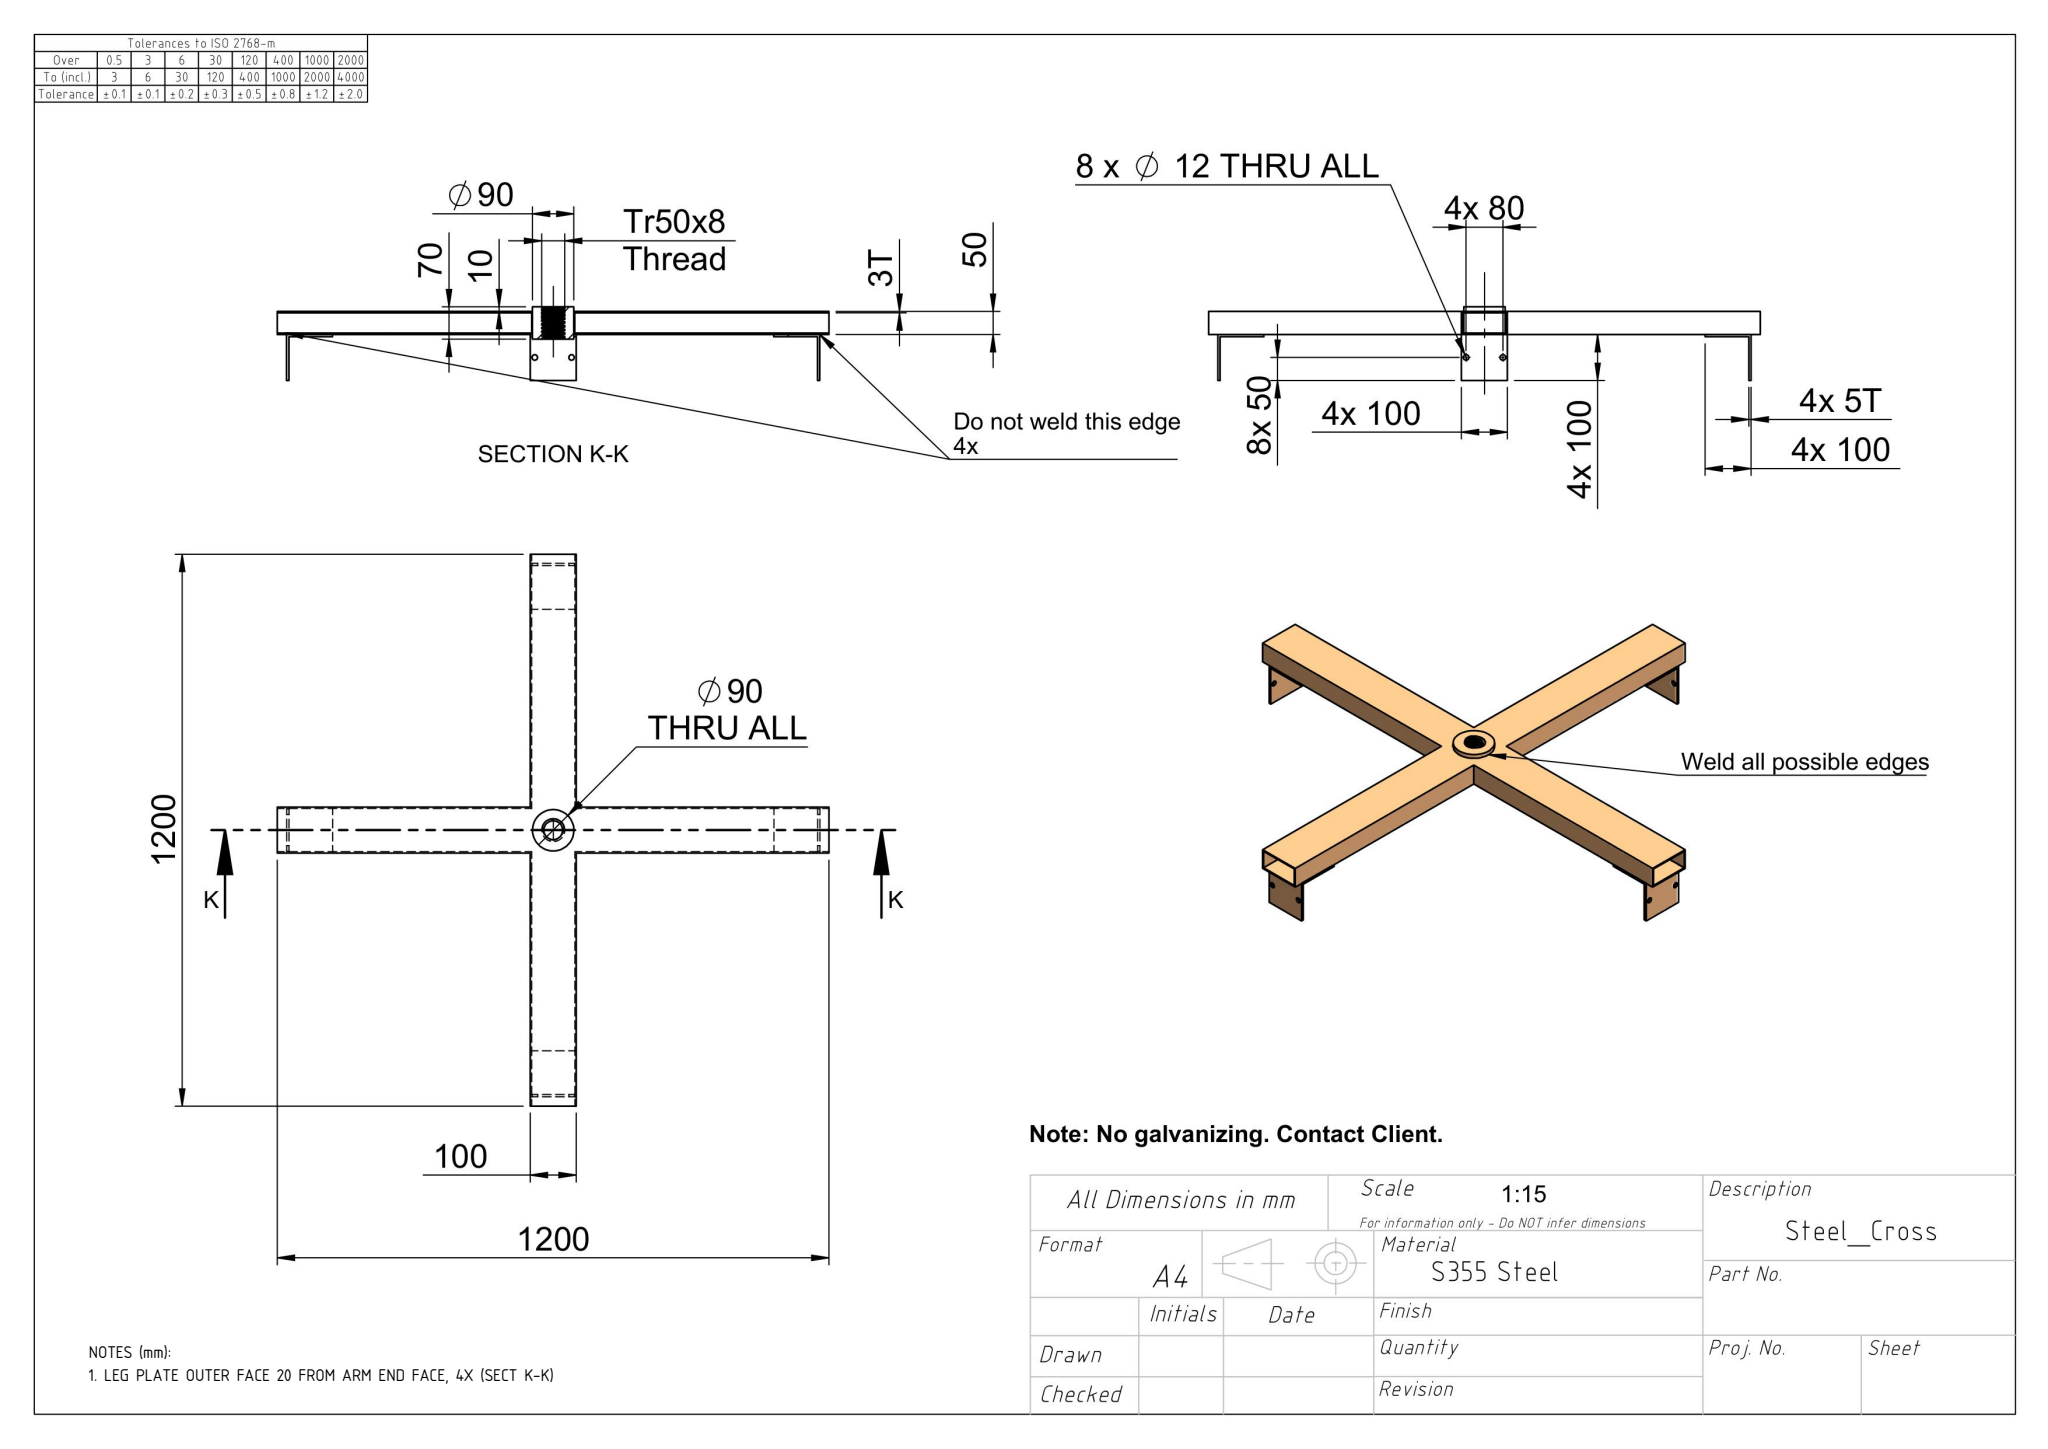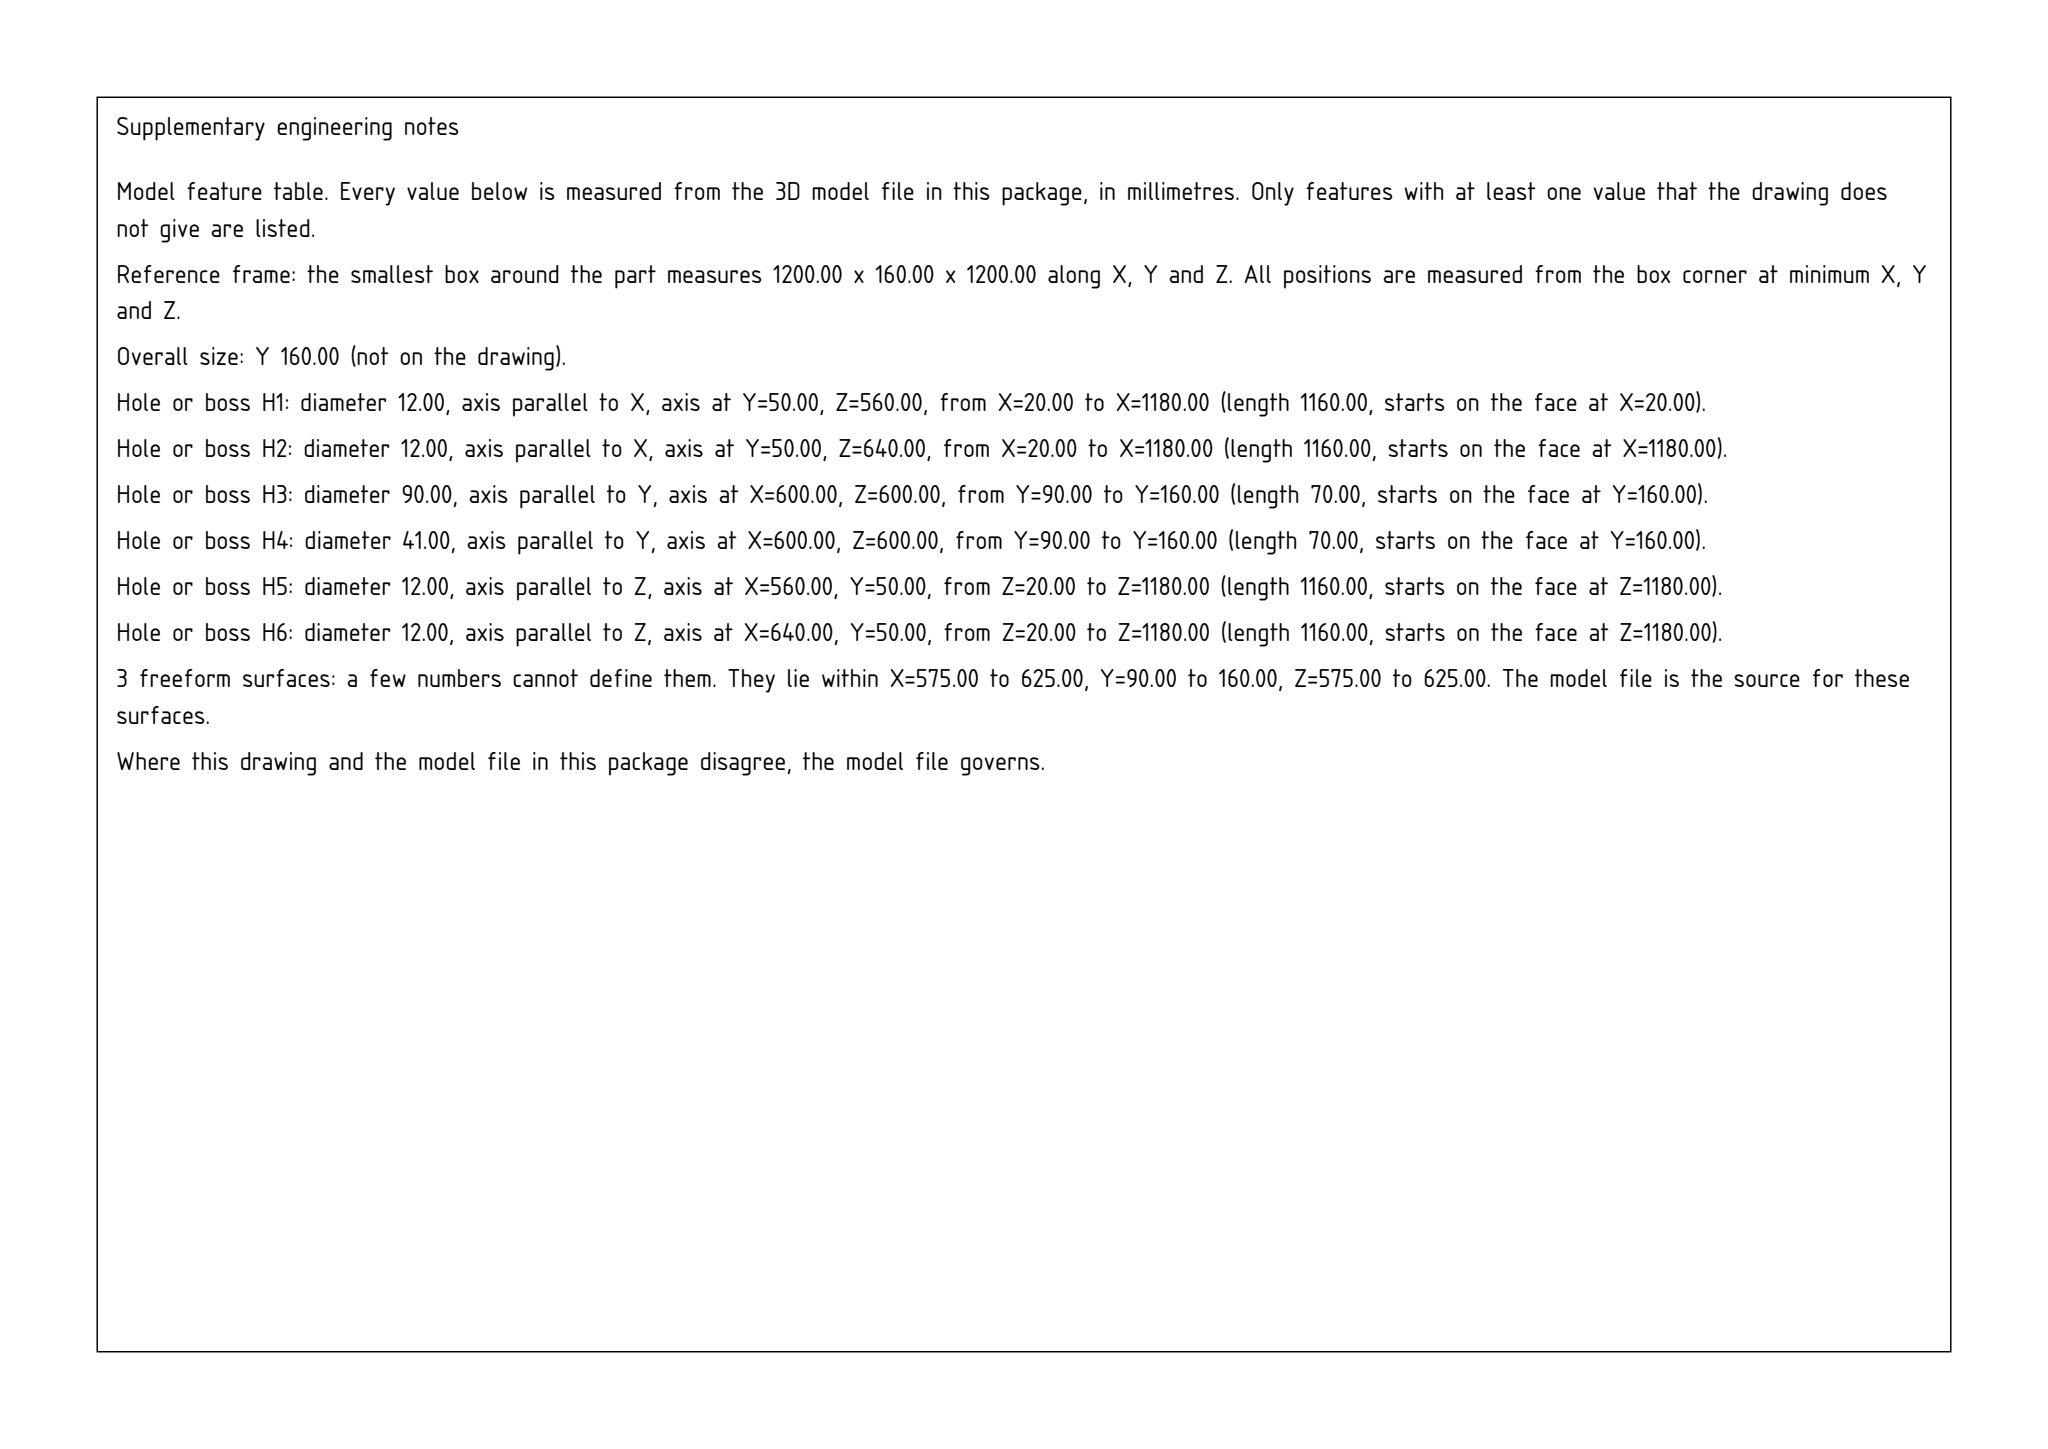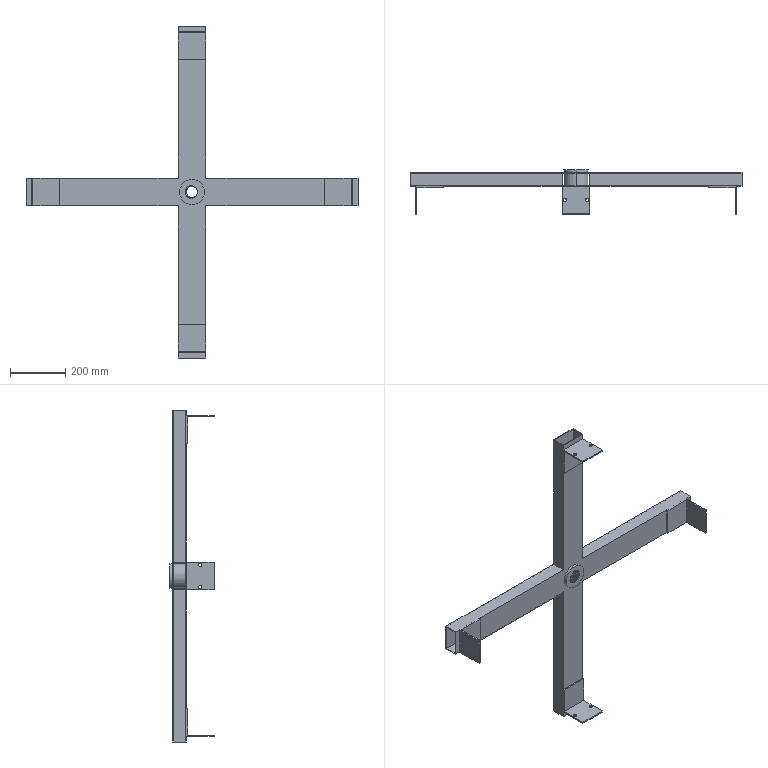Part | SolidWorks | mm | 1 solid | 94 faces | box 1200 x 160 x 1200 mm | volume 2639556 mm3 | plane 50 | cylinder 41 | spline 3 | commonest cylinder face diameters 41 x19 12 x16 90 x6
Drawing notes:
LEG PLATE OUTER FACE 20 FROM ARM END FACE, 4X (SECT K-K) | from the solid: x-planes 0 / 20 / 25 / 120 and 1200 / 1180 / 1175 / 1080; same in z: leg plate 5 thick set 20 in from each arm end, 100 flange